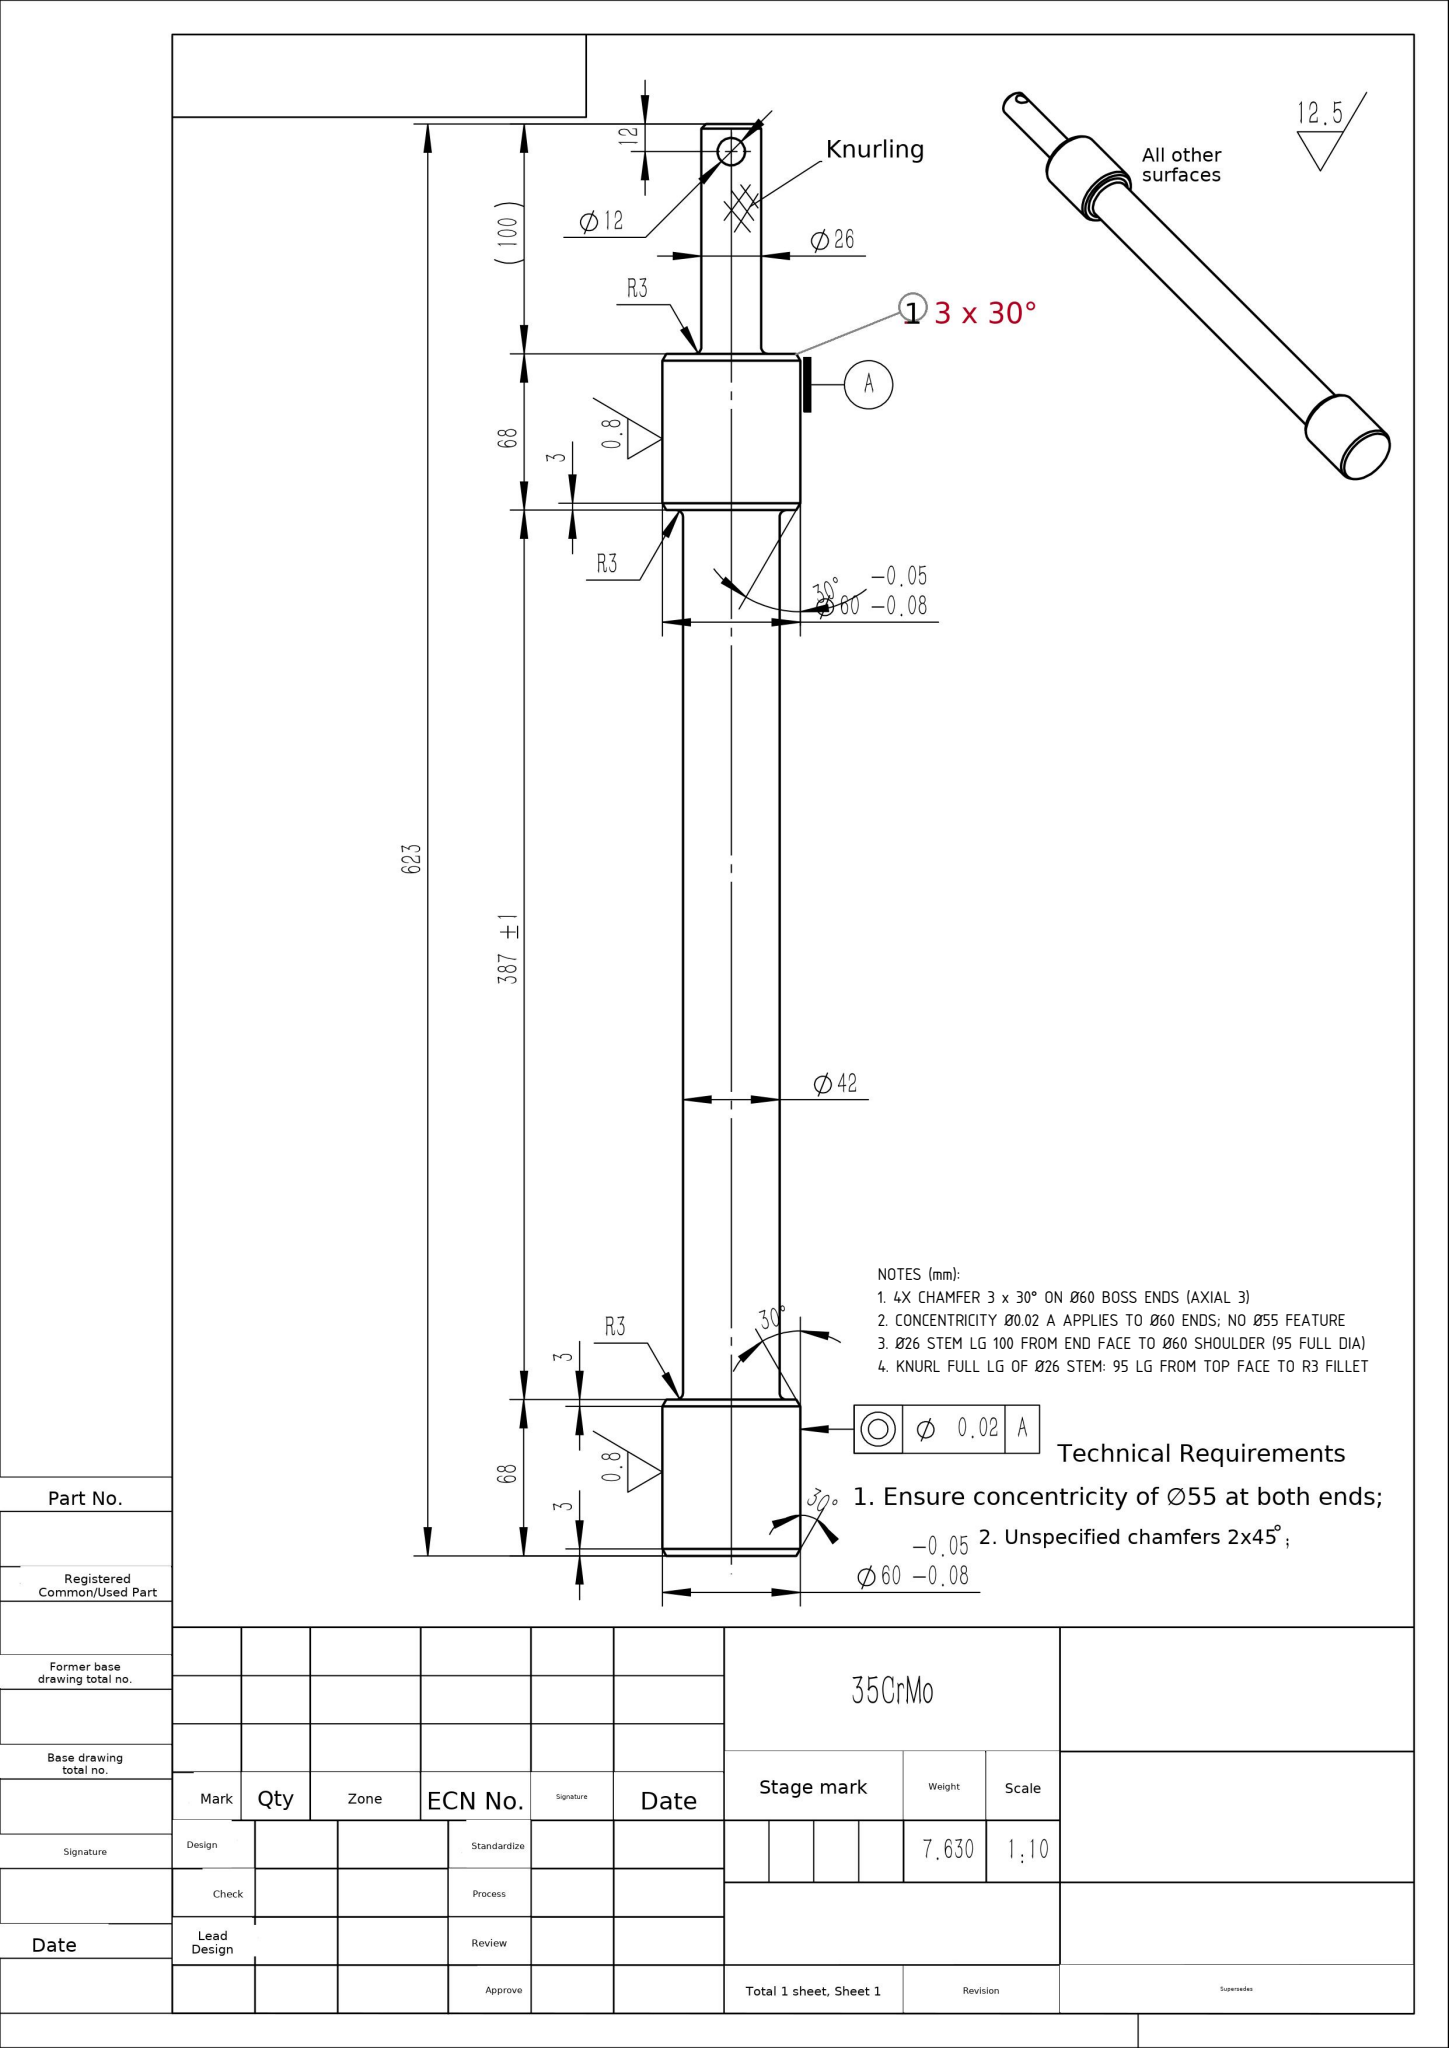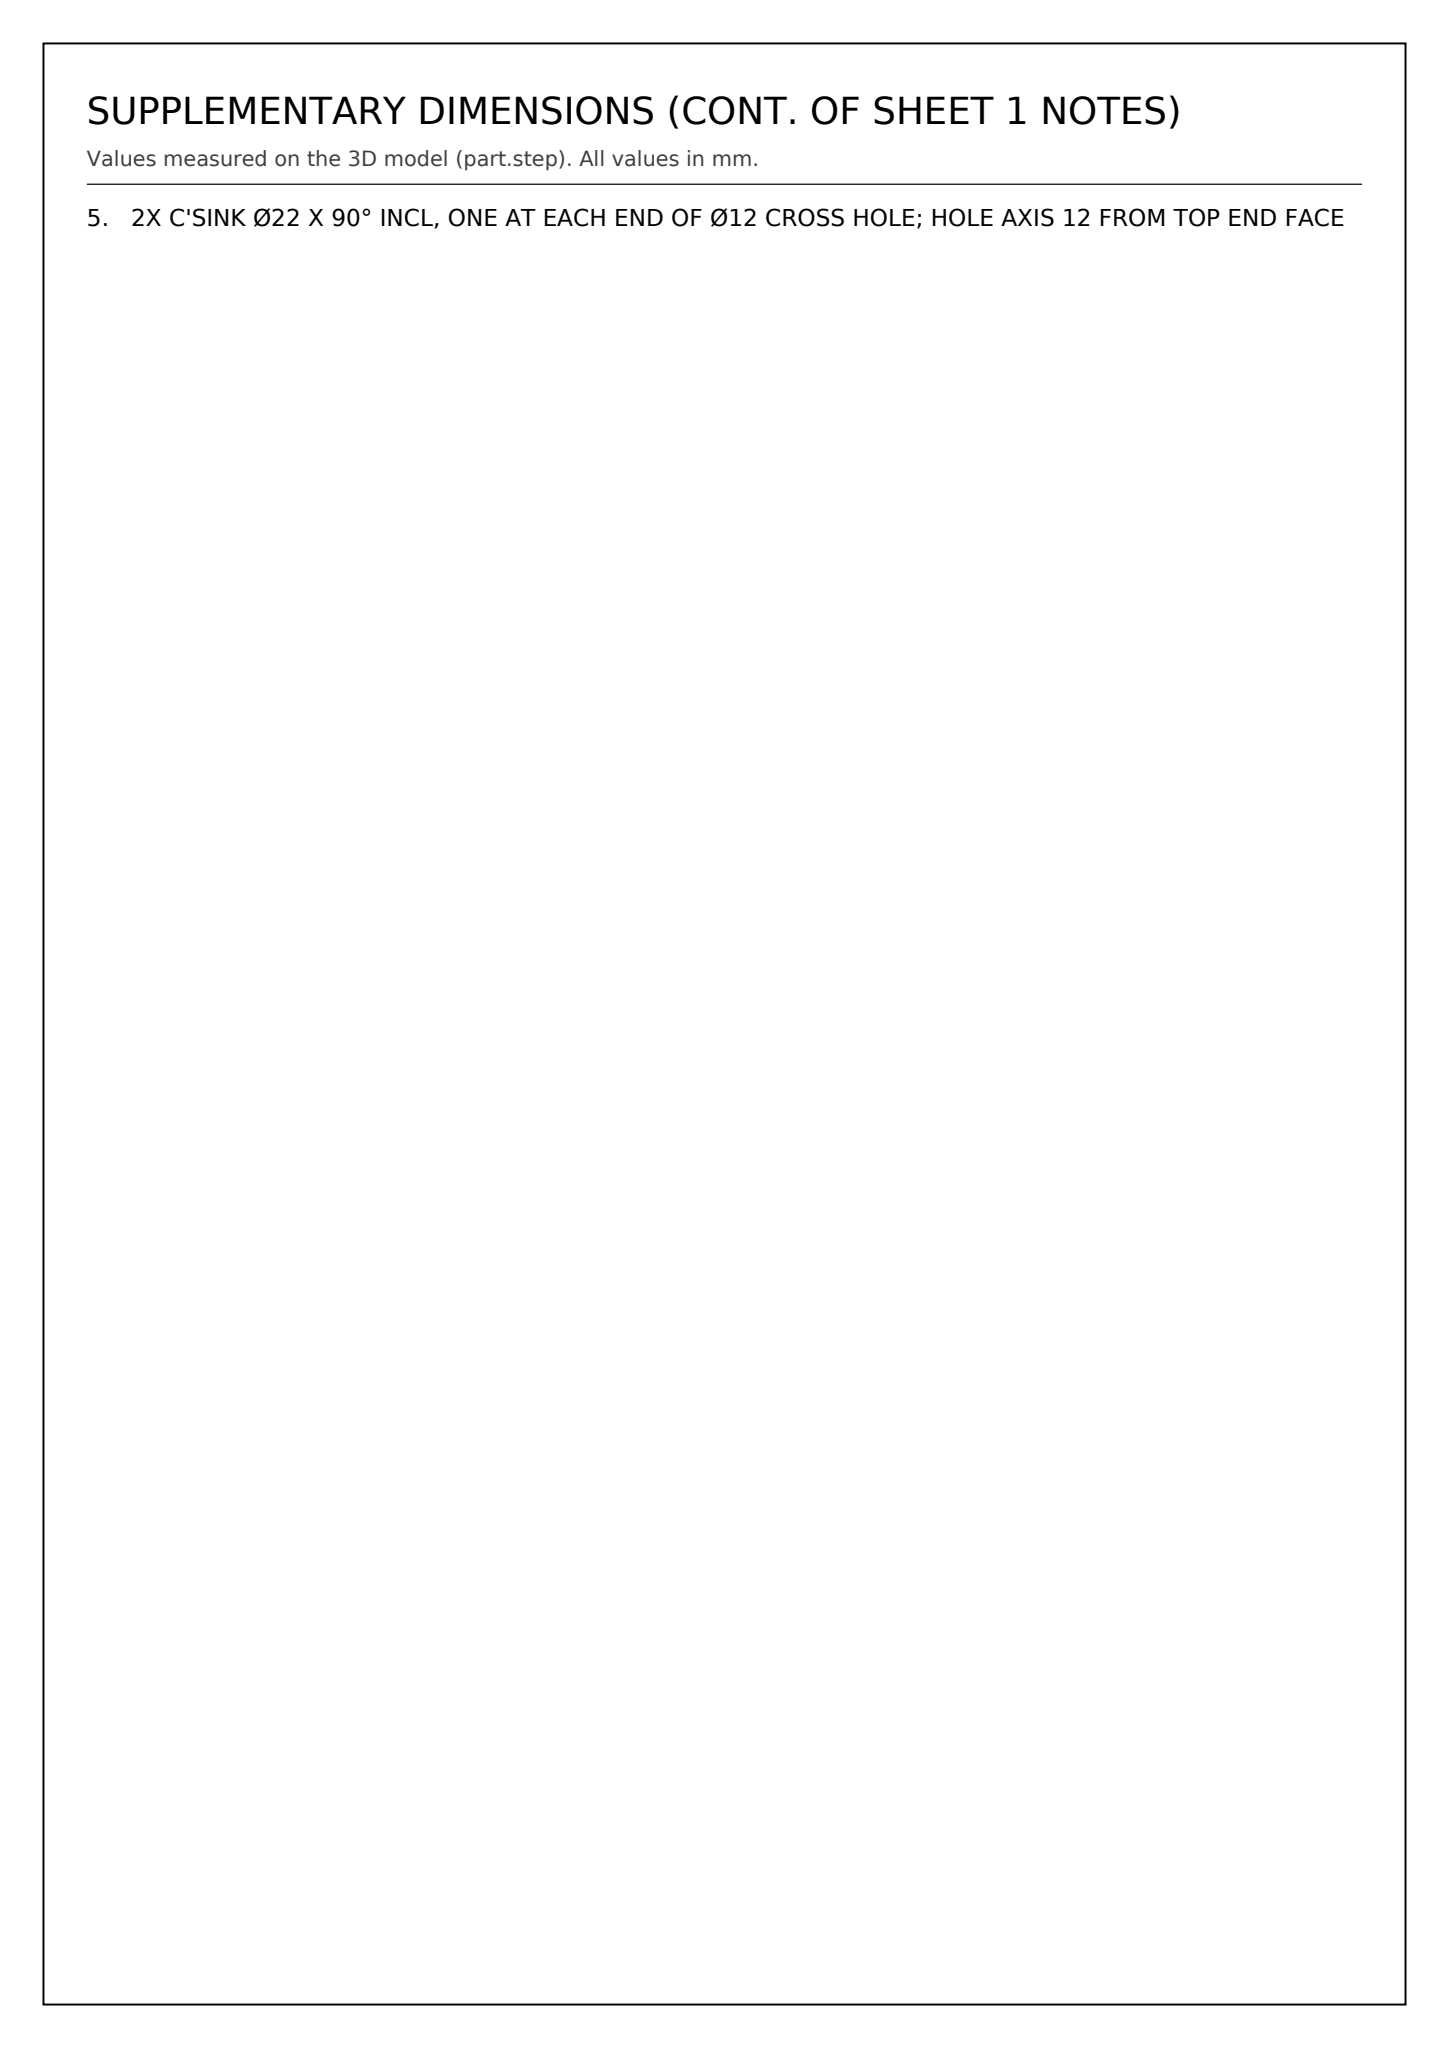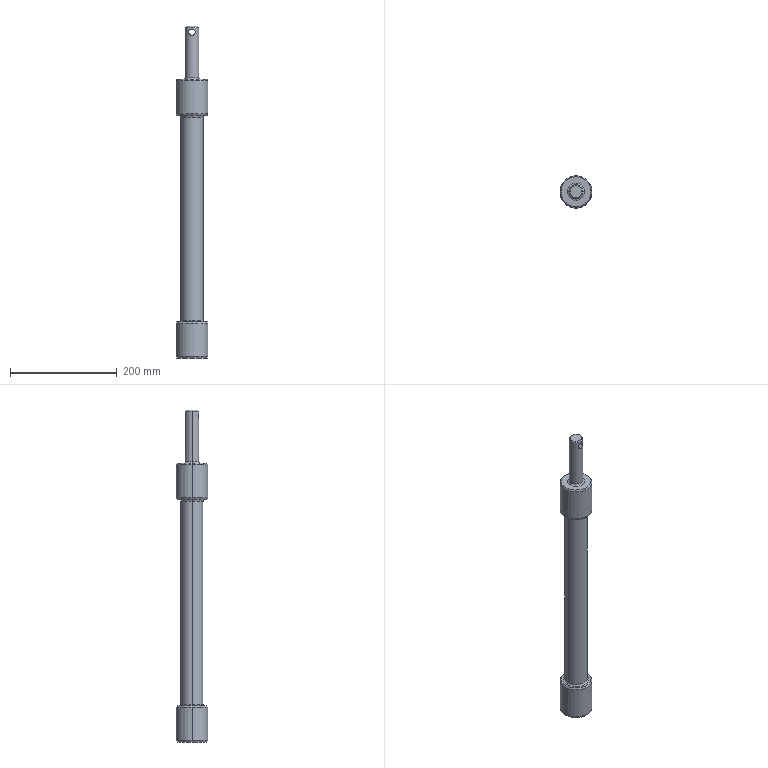Part | SolidWorks | mm | 1 solid | 31 faces | box 60 x 60 x 623 mm | volume 969546 mm3 | cylinder 10 | cone 10 | torus 6 | plane 5 | commonest cylinder face diameters 60 x4 12 x2 26 x2 42 x2
Drawing notes:
4X CHAMFER 3 x 30° ON Ø60 BOSS ENDS (AXIAL 3) | from the solid: cones 60° incl, ref dia 60.0 -> 56.536: 3.0 axial x 30° on all 4 Ø60 ends
CONCENTRICITY Ø0.02 A APPLIES TO Ø60 ENDS; NO Ø55 FEATURE | from the solid: only Ø60 cyls (L=62) at z=0-68 and z=455-523; no Ø55 cylinder in model
Ø26 STEM LG 100 FROM END FACE TO Ø60 SHOULDER (95 FULL DIA) | from the solid: Ø26 cyl L=95 between planes z=523 and z=623; R3 fillet at shoulder
KNURL FULL LG OF Ø26 STEM: 95 LG FROM TOP FACE TO R3 FILLET | from the solid: Cylinder Ø26 along z, length 95, from z=528 to top face z=623 (bbox z=623); R3 fillet at step to Ø60
2X C'SINK Ø22 X 90° INCL, ONE AT EACH END OF Ø12 CROSS HOLE; HOLE AXIS 12 FROM TOP END FACE | from the solid: cones[included_angle,ref_dia]=[90.0,22.0] count 2; cylinder dia 12 axis y at z=611 (623-611=12 from top face)
build123d program:
from build123d import *

# Parameters (mm, degrees)
SKETCH1_R               = 30
BOSS_EXTRUDE1_DEPTH     = 68
CHAMFER1_SIZE           = 3
CHAMFER1_SIZE2          = 1.732
CHAMFER2_SIZE           = 3
CHAMFER2_SIZE2          = 1.732
SKETCH2_R               = 21
BOSS_EXTRUDE2_DEPTH     = 387
BOSS_EXTRUDE3_START     = 68
SKETCH3_R               = 30
BOSS_EXTRUDE3_DEPTH     = 68
CHAMFER3_SIZE           = 3
CHAMFER3_SIZE2          = 1.732
CHAMFER4_SIZE           = 3
CHAMFER4_SIZE2          = 1.732
SKETCH4_R               = 13
BOSS_EXTRUDE4_DEPTH     = 100
CHAMFER5_SIZE           = 2
CUT_EXTRUDE1_DEPTH      = 457.974
CUT_EXTRUDE1_DEPTH_BACK = 457.974
SKETCH5_R               = 6
FILLET2_R               = 3
FILLET3_R               = 3


with BuildPart() as part:
    # Sketch1 → Boss-Extrude1 (new body)
    with BuildSketch(Plane.XY):
        Circle(SKETCH1_R)
    extrude(amount=BOSS_EXTRUDE1_DEPTH)

    # Chamfer1
    chamfer1_edges = [part.edges().sort_by_distance(p)[0] for p in [
        (-30, 0, 68),
    ]]
    chamfer1_side = [part.faces().sort_by_distance(p)[0] for p in [
        (-30, 0, 34),
    ]]
    chamfer(chamfer1_edges, length=CHAMFER1_SIZE, length2=CHAMFER1_SIZE2, reference=chamfer1_side[0])

    # Chamfer2
    chamfer2_edges = [part.edges().sort_by_distance(p)[0] for p in [
        (-30, 0, 0),
    ]]
    chamfer2_side = [part.faces().sort_by_distance(p)[0] for p in [
        (-30, 0, 32.5),
    ]]
    chamfer(chamfer2_edges, length=CHAMFER2_SIZE, length2=CHAMFER2_SIZE2, reference=chamfer2_side[0])

    # Sketch2 → Boss-Extrude2 (add)
    with BuildSketch(Plane(origin=(0, 0, 0), x_dir=(-1, 0, 0), z_dir=(0, 0, -1))):
        with Locations(Location((0, 0, 0), (0, 0, 180))):
            Circle(SKETCH2_R)
    extrude(amount=BOSS_EXTRUDE2_DEPTH)

    # Sketch3 → Boss-Extrude3 (add)
    with BuildSketch(Plane(origin=(0, 0, -387), x_dir=(-1, 0, 0), z_dir=(0, 0, -1)).offset(BOSS_EXTRUDE3_START)):
        with Locations(Location((0, 0, 0), (0, 0, 180))):
            Circle(SKETCH3_R)
    extrude(amount=-BOSS_EXTRUDE3_DEPTH)

    # Chamfer3
    chamfer3_edges = [part.edges().sort_by_distance(p)[0] for p in [
        (-30, 0, -387),
    ]]
    chamfer3_side = [part.faces().sort_by_distance(p)[0] for p in [
        (-30, 0, -421),
    ]]
    chamfer(chamfer3_edges, length=CHAMFER3_SIZE, length2=CHAMFER3_SIZE2, reference=chamfer3_side[0])

    # Chamfer4
    chamfer4_edges = [part.edges().sort_by_distance(p)[0] for p in [
        (-30, 0, -455),
    ]]
    chamfer4_side = [part.faces().sort_by_distance(p)[0] for p in [
        (-30, 0, -422.5),
    ]]
    chamfer(chamfer4_edges, length=CHAMFER4_SIZE, length2=CHAMFER4_SIZE2, reference=chamfer4_side[0])

    # Sketch4 → Boss-Extrude4 (add)
    with BuildSketch(Plane.XY.offset(68)):
        Circle(SKETCH4_R)
    extrude(amount=BOSS_EXTRUDE4_DEPTH)

    # Chamfer5
    chamfer5_edges = [part.edges().sort_by_distance(p)[0] for p in [
        (-13, 0, 168),
    ]]
    chamfer(chamfer5_edges, length=CHAMFER5_SIZE)

    # Sketch5 → Cut-Extrude1 (cut, two sides: drawn at the far end of the back side and taken through both)
    with BuildSketch(Plane(origin=(0, 0, 0), x_dir=(1, 0, 0), z_dir=(0, 1, 0)).offset(-CUT_EXTRUDE1_DEPTH_BACK)):
        with Locations(Location((0, -156, 0), (0, 0, 270))):
            Circle(SKETCH5_R)
    extrude(amount=CUT_EXTRUDE1_DEPTH + CUT_EXTRUDE1_DEPTH_BACK, mode=Mode.SUBTRACT)

    # Fillet2
    fillet2_edges = [part.edges().sort_by_distance(p)[0] for p in [
        (-13, 0, 68),
    ]]
    fillet(fillet2_edges, radius=FILLET2_R)

    # Fillet3
    fillet3_edges = [part.edges().sort_by_distance(p)[0] for p in [
        (-21, 0, 0),
        (-21, 0, -387),
    ]]
    fillet(fillet3_edges, radius=FILLET3_R)


solid = part.part